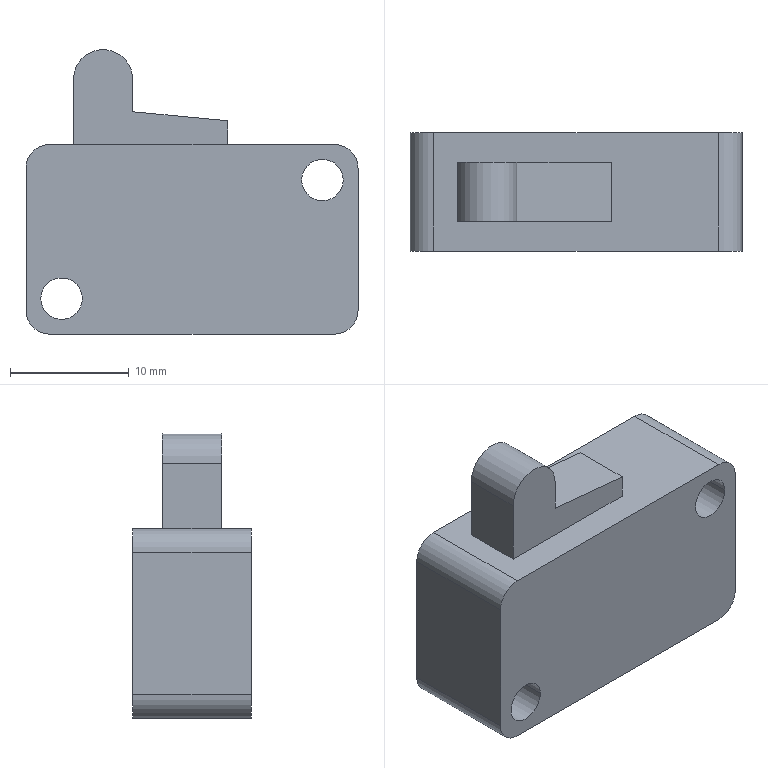Component | SolidWorks | 6G-LimitSwitch-1 | 1 solid | 21 faces | box 28 x 10 x 24 mm | volume 4535 mm3 | plane 12 | cylinder 9 | commonest cylinder face diameters 3.5 x4 4 x4 5 x1
build123d program:
from build123d import *

# Parameters (mm, degrees)
BOSS_EXTRUDE1_DEPTH = 5
SKETCH2_R           = 1.75
CUT_EXTRUDE1_DEPTH  = 10
SKETCH3_W           = 13
SKETCH3_H           = 5
BOSS_EXTRUDE2_DEPTH = 8
CUT_EXTRUDE2_DEPTH  = 8


with BuildPart() as part:
    # Sketch1 → Boss-Extrude1 (new, symmetric)
    with BuildSketch(Plane.XY):
        with BuildLine():
            Line((-12, -8), (12, -8))
            ThreePointArc((12, -8), (13.414, -7.414), (14, -6))
            Line((14, -6), (14, 6))
            ThreePointArc((14, 6), (13.414, 7.414), (12, 8))
            Line((12, 8), (-12, 8))
            ThreePointArc((-12, 8), (-13.414, 7.414), (-14, 6))
            Line((-14, 6), (-14, -6))
            ThreePointArc((-14, -6), (-13.414, -7.414), (-12, -8))
        make_face()
    extrude(amount=BOSS_EXTRUDE1_DEPTH, both=True)

    # Sketch2 → Cut-Extrude1 (cut)
    with BuildSketch(Plane.XY.offset(5)):
        with Locations((-11, 5)):
            Circle(SKETCH2_R)
        with Locations((11, -5)):
            Circle(SKETCH2_R)
    extrude(amount=-CUT_EXTRUDE1_DEPTH, mode=Mode.SUBTRACT)

    # Sketch3 → Boss-Extrude2 (add)
    with BuildSketch(Plane(origin=(0, 8, 0), x_dir=(1, 0, 0), z_dir=(0, 1, 0))):
        with Locations((3.5, 0)):
            Rectangle(SKETCH3_W, SKETCH3_H)
    extrude(amount=BOSS_EXTRUDE2_DEPTH)

    # Sketch4 → Cut-Extrude2 (cut)
    with BuildSketch(Plane.XY.offset(2.5)):
        with BuildLine():
            Line((-3, 10), (5, 10.762))
            Line((5, 10.762), (5, 13.5))
            ThreePointArc((5, 13.5), (7.5, 16), (10, 13.5))
            Line((10, 13.5), (11.275, 13.5))
            Line((11.275, 13.5), (11.275, 18.032))
            Line((11.275, 18.032), (-7.09, 18.279))
            Line((-7.09, 18.279), (-5.465, 11.216))
            Line((-5.465, 11.216), (-3, 10))
        make_face()
    extrude(amount=-CUT_EXTRUDE2_DEPTH, mode=Mode.SUBTRACT)


solid = part.part

# Placed as in the assembly
solid = solid.moved(Location((-161.85, 76, 22), (-90, 0, 180)))
STEP:
#1=COLOUR_RGB('',0.7922,0.8196,0.9333);
#2=FILL_AREA_STYLE_COLOUR('',#1);
#3=FILL_AREA_STYLE('',(#2));
#4=SURFACE_STYLE_FILL_AREA(#3);
#5=SURFACE_SIDE_STYLE('',(#4));
#6=SURFACE_STYLE_USAGE(.BOTH.,#5);
#7=PRESENTATION_STYLE_ASSIGNMENT((#6));
#8=CARTESIAN_POINT('',(-6.736,2.795,0.6693));
#9=VERTEX_POINT('',#8);
#10=CARTESIAN_POINT('',(-6.874,2.795,0.6693));
#11=VERTEX_POINT('',#10);
#12=CARTESIAN_POINT('',(-6.805,2.795,0.6693));
#13=DIRECTION('',(-0.,1.,0.));
#14=DIRECTION('',(-1.,0.,0.));
#15=AXIS2_PLACEMENT_3D('',#12,#13,#14);
#16=CIRCLE('',#15,0.0689);
#17=EDGE_CURVE('',#9,#11,#16,.T.);
#18=ORIENTED_EDGE('',*,*,#17,.F.);
#19=CARTESIAN_POINT('',(-6.736,3.189,0.6693));
#20=VERTEX_POINT('',#19);
#21=CARTESIAN_POINT('',(-6.736,2.795,0.6693));
#22=DIRECTION('',(-0.,1.,0.));
#23=VECTOR('',#22,39.37);
#24=LINE('',#21,#23);
#25=EDGE_CURVE('',#9,#20,#24,.T.);
#26=ORIENTED_EDGE('',*,*,#25,.T.);
#27=CARTESIAN_POINT('',(-6.874,3.189,0.6693));
#28=VERTEX_POINT('',#27);
#29=CARTESIAN_POINT('',(-6.805,3.189,0.6693));
#30=DIRECTION('',(-0.,1.,0.));
#31=DIRECTION('',(-1.,0.,0.));
#32=AXIS2_PLACEMENT_3D('',#29,#30,#31);
#33=CIRCLE('',#32,0.0689);
#34=EDGE_CURVE('',#20,#28,#33,.T.);
#35=ORIENTED_EDGE('',*,*,#34,.T.);
#36=CARTESIAN_POINT('',(-6.874,2.795,0.6693));
#37=DIRECTION('',(-0.,1.,0.));
#38=VECTOR('',#37,39.37);
#39=LINE('',#36,#38);
#40=EDGE_CURVE('',#11,#28,#39,.T.);
#41=ORIENTED_EDGE('',*,*,#40,.F.);
#42=EDGE_LOOP('',(#18,#26,#35,#41));
#43=FACE_OUTER_BOUND('',#42,.T.);
#44=CARTESIAN_POINT('',(-6.805,2.795,0.6693));
#45=DIRECTION('',(-0.,1.,0.));
#46=DIRECTION('',(-1.,0.,0.));
#47=AXIS2_PLACEMENT_3D('',#44,#45,#46);
#48=CYLINDRICAL_SURFACE('',#47,0.0689);
#49=ADVANCED_FACE('',(#43),#48,.F.);
#50=CARTESIAN_POINT('',(-5.87,2.795,1.063));
#51=VERTEX_POINT('',#50);
#52=CARTESIAN_POINT('',(-6.008,2.795,1.063));
#53=VERTEX_POINT('',#52);
#54=CARTESIAN_POINT('',(-5.939,2.795,1.063));
#55=DIRECTION('',(-0.,1.,0.));
#56=DIRECTION('',(-1.,0.,0.));
#57=AXIS2_PLACEMENT_3D('',#54,#55,#56);
#58=CIRCLE('',#57,0.0689);
#59=EDGE_CURVE('',#51,#53,#58,.T.);
#60=ORIENTED_EDGE('',*,*,#59,.F.);
#61=CARTESIAN_POINT('',(-5.87,3.189,1.063));
#62=VERTEX_POINT('',#61);
#63=CARTESIAN_POINT('',(-5.87,2.795,1.063));
#64=DIRECTION('',(-0.,1.,0.));
#65=VECTOR('',#64,39.37);
#66=LINE('',#63,#65);
#67=EDGE_CURVE('',#51,#62,#66,.T.);
#68=ORIENTED_EDGE('',*,*,#67,.T.);
#69=CARTESIAN_POINT('',(-6.008,3.189,1.063));
#70=VERTEX_POINT('',#69);
#71=CARTESIAN_POINT('',(-5.939,3.189,1.063));
#72=DIRECTION('',(-0.,1.,0.));
#73=DIRECTION('',(-1.,0.,0.));
#74=AXIS2_PLACEMENT_3D('',#71,#72,#73);
#75=CIRCLE('',#74,0.0689);
#76=EDGE_CURVE('',#62,#70,#75,.T.);
#77=ORIENTED_EDGE('',*,*,#76,.T.);
#78=CARTESIAN_POINT('',(-6.008,2.795,1.063));
#79=DIRECTION('',(-0.,1.,0.));
#80=VECTOR('',#79,39.37);
#81=LINE('',#78,#80);
#82=EDGE_CURVE('',#53,#70,#81,.T.);
#83=ORIENTED_EDGE('',*,*,#82,.F.);
#84=EDGE_LOOP('',(#60,#68,#77,#83));
#85=FACE_OUTER_BOUND('',#84,.T.);
#86=CARTESIAN_POINT('',(-5.939,2.795,1.063));
#87=DIRECTION('',(-0.,1.,0.));
#88=DIRECTION('',(-1.,0.,0.));
#89=AXIS2_PLACEMENT_3D('',#86,#87,#88);
#90=CYLINDRICAL_SURFACE('',#89,0.0689);
#91=ADVANCED_FACE('',(#85),#90,.F.);
#92=CARTESIAN_POINT('',(-6.844,2.795,1.181));
#93=VERTEX_POINT('',#92);
#94=CARTESIAN_POINT('',(-5.9,2.795,1.181));
#95=VERTEX_POINT('',#94);
#96=CARTESIAN_POINT('',(-5.9,2.795,1.181));
#97=DIRECTION('',(1.,0.,0.));
#98=VECTOR('',#97,39.37);
#99=LINE('',#96,#98);
#100=EDGE_CURVE('',#93,#95,#99,.T.);
#101=ORIENTED_EDGE('',*,*,#100,.T.);
#102=CARTESIAN_POINT('',(-5.9,3.189,1.181));
#103=VERTEX_POINT('',#102);
#104=CARTESIAN_POINT('',(-5.9,3.189,1.181));
#105=DIRECTION('',(0.,-1.,-0.));
#106=VECTOR('',#105,39.37);
#107=LINE('',#104,#106);
#108=EDGE_CURVE('',#103,#95,#107,.T.);
#109=ORIENTED_EDGE('',*,*,#108,.F.);
#110=CARTESIAN_POINT('',(-6.844,3.189,1.181));
#111=VERTEX_POINT('',#110);
#112=CARTESIAN_POINT('',(-5.9,3.189,1.181));
#113=DIRECTION('',(1.,0.,0.));
#114=VECTOR('',#113,39.37);
#115=LINE('',#112,#114);
#116=EDGE_CURVE('',#111,#103,#115,.T.);
#117=ORIENTED_EDGE('',*,*,#116,.F.);
#118=CARTESIAN_POINT('',(-6.844,3.189,1.181));
#119=DIRECTION('',(0.,-1.,-0.));
#120=VECTOR('',#119,39.37);
#121=LINE('',#118,#120);
#122=EDGE_CURVE('',#111,#93,#121,.T.);
#123=ORIENTED_EDGE('',*,*,#122,.T.);
#124=EDGE_LOOP('',(#101,#109,#117,#123));
#125=FACE_OUTER_BOUND('',#124,.T.);
#126=CARTESIAN_POINT('',(-6.766,2.894,1.181));
#127=VERTEX_POINT('',#126);
#128=CARTESIAN_POINT('',(-6.254,2.894,1.181));
#129=VERTEX_POINT('',#128);
#130=CARTESIAN_POINT('',(-6.766,2.894,1.181));
#131=DIRECTION('',(1.,0.,0.));
#132=VECTOR('',#131,39.37);
#133=LINE('',#130,#132);
#134=EDGE_CURVE('',#127,#129,#133,.T.);
#135=ORIENTED_EDGE('',*,*,#134,.F.);
#136=CARTESIAN_POINT('',(-6.766,3.091,1.181));
#137=VERTEX_POINT('',#136);
#138=CARTESIAN_POINT('',(-6.766,3.091,1.181));
#139=DIRECTION('',(0.,-1.,-0.));
#140=VECTOR('',#139,39.37);
#141=LINE('',#138,#140);
#142=EDGE_CURVE('',#137,#127,#141,.T.);
#143=ORIENTED_EDGE('',*,*,#142,.F.);
#144=CARTESIAN_POINT('',(-6.254,3.091,1.181));
#145=VERTEX_POINT('',#144);
#146=CARTESIAN_POINT('',(-6.766,3.091,1.181));
#147=DIRECTION('',(-1.,-0.,-0.));
#148=VECTOR('',#147,39.37);
#149=LINE('',#146,#148);
#150=EDGE_CURVE('',#145,#137,#149,.T.);
#151=ORIENTED_EDGE('',*,*,#150,.F.);
#152=CARTESIAN_POINT('',(-6.254,3.091,1.181));
#153=DIRECTION('',(-0.,1.,0.));
#154=VECTOR('',#153,39.37);
#155=LINE('',#152,#154);
#156=EDGE_CURVE('',#129,#145,#155,.T.);
#157=ORIENTED_EDGE('',*,*,#156,.F.);
#158=EDGE_LOOP('',(#135,#143,#151,#157));
#159=FACE_BOUND('',#158,.T.);
#160=CARTESIAN_POINT('',(-5.9,3.189,1.181));
#161=DIRECTION('',(0.,0.,-1.));
#162=DIRECTION('',(0.,-1.,-0.));
#163=AXIS2_PLACEMENT_3D('',#160,#161,#162);
#164=PLANE('',#163);
#165=ADVANCED_FACE('',(#125,#159),#164,.F.);
#166=CARTESIAN_POINT('',(-5.821,2.795,0.6299));
#167=VERTEX_POINT('',#166);
#168=CARTESIAN_POINT('',(-5.9,2.795,0.5512));
#169=VERTEX_POINT('',#168);
#170=CARTESIAN_POINT('',(-5.9,2.795,0.6299));
#171=DIRECTION('',(-0.,1.,0.));
#172=DIRECTION('',(1.,0.,0.));
#173=AXIS2_PLACEMENT_3D('',#170,#171,#172);
#174=CIRCLE('',#173,0.07874);
#175=EDGE_CURVE('',#167,#169,#174,.T.);
#176=ORIENTED_EDGE('',*,*,#175,.T.);
#177=CARTESIAN_POINT('',(-5.9,3.189,0.5512));
#178=VERTEX_POINT('',#177);
#179=CARTESIAN_POINT('',(-5.9,3.189,0.5512));
#180=DIRECTION('',(0.,-1.,-0.));
#181=VECTOR('',#180,39.37);
#182=LINE('',#179,#181);
#183=EDGE_CURVE('',#178,#169,#182,.T.);
#184=ORIENTED_EDGE('',*,*,#183,.F.);
#185=CARTESIAN_POINT('',(-5.821,3.189,0.6299));
#186=VERTEX_POINT('',#185);
#187=CARTESIAN_POINT('',(-5.9,3.189,0.6299));
#188=DIRECTION('',(-0.,1.,0.));
#189=DIRECTION('',(1.,0.,0.));
#190=AXIS2_PLACEMENT_3D('',#187,#188,#189);
#191=CIRCLE('',#190,0.07874);
#192=EDGE_CURVE('',#186,#178,#191,.T.);
#193=ORIENTED_EDGE('',*,*,#192,.F.);
#194=CARTESIAN_POINT('',(-5.821,3.189,0.6299));
#195=DIRECTION('',(0.,-1.,-0.));
#196=VECTOR('',#195,39.37);
#197=LINE('',#194,#196);
#198=EDGE_CURVE('',#186,#167,#197,.T.);
#199=ORIENTED_EDGE('',*,*,#198,.T.);
#200=EDGE_LOOP('',(#176,#184,#193,#199));
#201=FACE_OUTER_BOUND('',#200,.T.);
#202=CARTESIAN_POINT('',(-5.9,3.189,0.6299));
#203=DIRECTION('',(0.,-1.,-0.));
#204=DIRECTION('',(1.,0.,0.));
#205=AXIS2_PLACEMENT_3D('',#202,#203,#204);
#206=CYLINDRICAL_SURFACE('',#205,0.07874);
#207=ADVANCED_FACE('',(#201),#206,.T.);
#208=CARTESIAN_POINT('',(-6.844,2.795,0.5512));
#209=VERTEX_POINT('',#208);
#210=CARTESIAN_POINT('',(-5.9,2.795,0.5512));
#211=DIRECTION('',(-1.,-0.,-0.));
#212=VECTOR('',#211,39.37);
#213=LINE('',#210,#212);
#214=EDGE_CURVE('',#169,#209,#213,.T.);
#215=ORIENTED_EDGE('',*,*,#214,.T.);
#216=CARTESIAN_POINT('',(-6.844,3.189,0.5512));
#217=VERTEX_POINT('',#216);
#218=CARTESIAN_POINT('',(-6.844,3.189,0.5512));
#219=DIRECTION('',(0.,-1.,-0.));
#220=VECTOR('',#219,39.37);
#221=LINE('',#218,#220);
#222=EDGE_CURVE('',#217,#209,#221,.T.);
#223=ORIENTED_EDGE('',*,*,#222,.F.);
#224=CARTESIAN_POINT('',(-5.9,3.189,0.5512));
#225=DIRECTION('',(-1.,-0.,-0.));
#226=VECTOR('',#225,39.37);
#227=LINE('',#224,#226);
#228=EDGE_CURVE('',#178,#217,#227,.T.);
#229=ORIENTED_EDGE('',*,*,#228,.F.);
#230=ORIENTED_EDGE('',*,*,#183,.T.);
#231=EDGE_LOOP('',(#215,#223,#229,#230));
#232=FACE_OUTER_BOUND('',#231,.T.);
#233=CARTESIAN_POINT('',(-5.9,3.189,0.5512));
#234=DIRECTION('',(-0.,-0.,1.));
#235=DIRECTION('',(-0.,1.,0.));
#236=AXIS2_PLACEMENT_3D('',#233,#234,#235);
#237=PLANE('',#236);
#238=ADVANCED_FACE('',(#232),#237,.F.);
#239=CARTESIAN_POINT('',(-6.923,2.795,0.6299));
#240=VERTEX_POINT('',#239);
#241=CARTESIAN_POINT('',(-6.844,2.795,0.6299));
#242=DIRECTION('',(-0.,1.,0.));
#243=DIRECTION('',(-1.,0.,0.));
#244=AXIS2_PLACEMENT_3D('',#241,#242,#243);
#245=CIRCLE('',#244,0.07874);
#246=EDGE_CURVE('',#209,#240,#245,.T.);
#247=ORIENTED_EDGE('',*,*,#246,.T.);
#248=CARTESIAN_POINT('',(-6.923,3.189,0.6299));
#249=VERTEX_POINT('',#248);
#250=CARTESIAN_POINT('',(-6.923,3.189,0.6299));
#251=DIRECTION('',(0.,-1.,-0.));
#252=VECTOR('',#251,39.37);
#253=LINE('',#250,#252);
#254=EDGE_CURVE('',#249,#240,#253,.T.);
#255=ORIENTED_EDGE('',*,*,#254,.F.);
#256=CARTESIAN_POINT('',(-6.844,3.189,0.6299));
#257=DIRECTION('',(-0.,1.,0.));
#258=DIRECTION('',(-1.,0.,0.));
#259=AXIS2_PLACEMENT_3D('',#256,#257,#258);
#260=CIRCLE('',#259,0.07874);
#261=EDGE_CURVE('',#217,#249,#260,.T.);
#262=ORIENTED_EDGE('',*,*,#261,.F.);
#263=ORIENTED_EDGE('',*,*,#222,.T.);
#264=EDGE_LOOP('',(#247,#255,#262,#263));
#265=FACE_OUTER_BOUND('',#264,.T.);
#266=CARTESIAN_POINT('',(-6.844,3.189,0.6299));
#267=DIRECTION('',(0.,-1.,-0.));
#268=DIRECTION('',(1.,0.,0.));
#269=AXIS2_PLACEMENT_3D('',#266,#267,#268);
#270=CYLINDRICAL_SURFACE('',#269,0.07874);
#271=ADVANCED_FACE('',(#265),#270,.T.);
#272=CARTESIAN_POINT('',(-6.923,2.795,1.102));
#273=VERTEX_POINT('',#272);
#274=CARTESIAN_POINT('',(-6.923,2.795,0.6299));
#275=DIRECTION('',(-0.,-0.,1.));
#276=VECTOR('',#275,39.37);
#277=LINE('',#274,#276);
#278=EDGE_CURVE('',#240,#273,#277,.T.);
#279=ORIENTED_EDGE('',*,*,#278,.T.);
#280=CARTESIAN_POINT('',(-6.923,3.189,1.102));
#281=VERTEX_POINT('',#280);
#282=CARTESIAN_POINT('',(-6.923,3.189,1.102));
#283=DIRECTION('',(0.,-1.,-0.));
#284=VECTOR('',#283,39.37);
#285=LINE('',#282,#284);
#286=EDGE_CURVE('',#281,#273,#285,.T.);
#287=ORIENTED_EDGE('',*,*,#286,.F.);
#288=CARTESIAN_POINT('',(-6.923,3.189,0.6299));
#289=DIRECTION('',(-0.,-0.,1.));
#290=VECTOR('',#289,39.37);
#291=LINE('',#288,#290);
#292=EDGE_CURVE('',#249,#281,#291,.T.);
#293=ORIENTED_EDGE('',*,*,#292,.F.);
#294=ORIENTED_EDGE('',*,*,#254,.T.);
#295=EDGE_LOOP('',(#279,#287,#293,#294));
#296=FACE_OUTER_BOUND('',#295,.T.);
#297=CARTESIAN_POINT('',(-6.923,3.189,0.6299));
#298=DIRECTION('',(1.,0.,0.));
#299=DIRECTION('',(-0.,1.,0.));
#300=AXIS2_PLACEMENT_3D('',#297,#298,#299);
#301=PLANE('',#300);
#302=ADVANCED_FACE('',(#296),#301,.F.);
#303=CARTESIAN_POINT('',(-6.844,2.795,1.102));
#304=DIRECTION('',(-0.,1.,0.));
#305=DIRECTION('',(1.,0.,0.));
#306=AXIS2_PLACEMENT_3D('',#303,#304,#305);
#307=CIRCLE('',#306,0.07874);
#308=EDGE_CURVE('',#273,#93,#307,.T.);
#309=ORIENTED_EDGE('',*,*,#308,.T.);
#310=ORIENTED_EDGE('',*,*,#122,.F.);
#311=CARTESIAN_POINT('',(-6.844,3.189,1.102));
#312=DIRECTION('',(-0.,1.,0.));
#313=DIRECTION('',(1.,0.,0.));
#314=AXIS2_PLACEMENT_3D('',#311,#312,#313);
#315=CIRCLE('',#314,0.07874);
#316=EDGE_CURVE('',#281,#111,#315,.T.);
#317=ORIENTED_EDGE('',*,*,#316,.F.);
#318=ORIENTED_EDGE('',*,*,#286,.T.);
#319=EDGE_LOOP('',(#309,#310,#317,#318));
#320=FACE_OUTER_BOUND('',#319,.T.);
#321=CARTESIAN_POINT('',(-6.844,3.189,1.102));
#322=DIRECTION('',(0.,-1.,-0.));
#323=DIRECTION('',(1.,0.,0.));
#324=AXIS2_PLACEMENT_3D('',#321,#322,#323);
#325=CYLINDRICAL_SURFACE('',#324,0.07874);
#326=ADVANCED_FACE('',(#320),#325,.T.);
#327=CARTESIAN_POINT('',(-5.821,2.795,1.102));
#328=VERTEX_POINT('',#327);
#329=CARTESIAN_POINT('',(-5.9,2.795,1.102));
#330=DIRECTION('',(-0.,1.,0.));
#331=DIRECTION('',(1.,0.,0.));
#332=AXIS2_PLACEMENT_3D('',#329,#330,#331);
#333=CIRCLE('',#332,0.07874);
#334=EDGE_CURVE('',#95,#328,#333,.T.);
#335=ORIENTED_EDGE('',*,*,#334,.T.);
#336=CARTESIAN_POINT('',(-5.821,3.189,1.102));
#337=VERTEX_POINT('',#336);
#338=CARTESIAN_POINT('',(-5.821,3.189,1.102));
#339=DIRECTION('',(0.,-1.,-0.));
#340=VECTOR('',#339,39.37);
#341=LINE('',#338,#340);
#342=EDGE_CURVE('',#337,#328,#341,.T.);
#343=ORIENTED_EDGE('',*,*,#342,.F.);
#344=CARTESIAN_POINT('',(-5.9,3.189,1.102));
#345=DIRECTION('',(-0.,1.,0.));
#346=DIRECTION('',(1.,0.,0.));
#347=AXIS2_PLACEMENT_3D('',#344,#345,#346);
#348=CIRCLE('',#347,0.07874);
#349=EDGE_CURVE('',#103,#337,#348,.T.);
#350=ORIENTED_EDGE('',*,*,#349,.F.);
#351=ORIENTED_EDGE('',*,*,#108,.T.);
#352=EDGE_LOOP('',(#335,#343,#350,#351));
#353=FACE_OUTER_BOUND('',#352,.T.);
#354=CARTESIAN_POINT('',(-5.9,3.189,1.102));
#355=DIRECTION('',(0.,-1.,-0.));
#356=DIRECTION('',(1.,0.,0.));
#357=AXIS2_PLACEMENT_3D('',#354,#355,#356);
#358=CYLINDRICAL_SURFACE('',#357,0.07874);
#359=ADVANCED_FACE('',(#353),#358,.T.);
#360=CARTESIAN_POINT('',(-5.821,2.795,0.6299));
#361=DIRECTION('',(0.,0.,-1.));
#362=VECTOR('',#361,39.37);
#363=LINE('',#360,#362);
#364=EDGE_CURVE('',#328,#167,#363,.T.);
#365=ORIENTED_EDGE('',*,*,#364,.T.);
#366=ORIENTED_EDGE('',*,*,#198,.F.);
#367=CARTESIAN_POINT('',(-5.821,3.189,0.6299));
#368=DIRECTION('',(0.,0.,-1.));
#369=VECTOR('',#368,39.37);
#370=LINE('',#367,#369);
#371=EDGE_CURVE('',#337,#186,#370,.T.);
#372=ORIENTED_EDGE('',*,*,#371,.F.);
#373=ORIENTED_EDGE('',*,*,#342,.T.);
#374=EDGE_LOOP('',(#365,#366,#372,#373));
#375=FACE_OUTER_BOUND('',#374,.T.);
#376=CARTESIAN_POINT('',(-5.821,3.189,0.6299));
#377=DIRECTION('',(-1.,-0.,-0.));
#378=DIRECTION('',(0.,-1.,-0.));
#379=AXIS2_PLACEMENT_3D('',#376,#377,#378);
#380=PLANE('',#379);
#381=ADVANCED_FACE('',(#375),#380,.F.);
#382=CARTESIAN_POINT('',(-6.805,3.189,0.6693));
#383=DIRECTION('',(-0.,1.,0.));
#384=DIRECTION('',(-1.,0.,0.));
#385=AXIS2_PLACEMENT_3D('',#382,#383,#384);
#386=CIRCLE('',#385,0.0689);
#387=EDGE_CURVE('',#28,#20,#386,.T.);
#388=ORIENTED_EDGE('',*,*,#387,.F.);
#389=ORIENTED_EDGE('',*,*,#34,.F.);
#390=EDGE_LOOP('',(#388,#389));
#391=FACE_BOUND('',#390,.T.);
#392=CARTESIAN_POINT('',(-5.939,3.189,1.063));
#393=DIRECTION('',(-0.,1.,0.));
#394=DIRECTION('',(-1.,0.,0.));
#395=AXIS2_PLACEMENT_3D('',#392,#393,#394);
#396=CIRCLE('',#395,0.0689);
#397=EDGE_CURVE('',#70,#62,#396,.T.);
#398=ORIENTED_EDGE('',*,*,#397,.F.);
#399=ORIENTED_EDGE('',*,*,#76,.F.);
#400=EDGE_LOOP('',(#398,#399));
#401=FACE_BOUND('',#400,.T.);
#402=ORIENTED_EDGE('',*,*,#192,.T.);
#403=ORIENTED_EDGE('',*,*,#228,.T.);
#404=ORIENTED_EDGE('',*,*,#261,.T.);
#405=ORIENTED_EDGE('',*,*,#292,.T.);
#406=ORIENTED_EDGE('',*,*,#316,.T.);
#407=ORIENTED_EDGE('',*,*,#116,.T.);
#408=ORIENTED_EDGE('',*,*,#349,.T.);
#409=ORIENTED_EDGE('',*,*,#371,.T.);
#410=EDGE_LOOP('',(#402,#403,#404,#405,#406,#407,#408,#409));
#411=FACE_OUTER_BOUND('',#410,.T.);
#412=CARTESIAN_POINT('',(-5.9,3.189,0.6299));
#413=DIRECTION('',(0.,-1.,-0.));
#414=DIRECTION('',(1.,0.,0.));
#415=AXIS2_PLACEMENT_3D('',#412,#413,#414);
#416=PLANE('',#415);
#417=ADVANCED_FACE('',(#391,#401,#411),#416,.F.);
#418=CARTESIAN_POINT('',(-6.805,2.795,0.6693));
#419=DIRECTION('',(-0.,1.,0.));
#420=DIRECTION('',(-1.,0.,0.));
#421=AXIS2_PLACEMENT_3D('',#418,#419,#420);
#422=CIRCLE('',#421,0.0689);
#423=EDGE_CURVE('',#11,#9,#422,.T.);
#424=ORIENTED_EDGE('',*,*,#423,.T.);
#425=ORIENTED_EDGE('',*,*,#17,.T.);
#426=EDGE_LOOP('',(#424,#425));
#427=FACE_BOUND('',#426,.T.);
#428=CARTESIAN_POINT('',(-5.939,2.795,1.063));
#429=DIRECTION('',(-0.,1.,0.));
#430=DIRECTION('',(-1.,0.,0.));
#431=AXIS2_PLACEMENT_3D('',#428,#429,#430);
#432=CIRCLE('',#431,0.0689);
#433=EDGE_CURVE('',#53,#51,#432,.T.);
#434=ORIENTED_EDGE('',*,*,#433,.T.);
#435=ORIENTED_EDGE('',*,*,#59,.T.);
#436=EDGE_LOOP('',(#434,#435));
#437=FACE_BOUND('',#436,.T.);
#438=ORIENTED_EDGE('',*,*,#175,.F.);
#439=ORIENTED_EDGE('',*,*,#364,.F.);
#440=ORIENTED_EDGE('',*,*,#334,.F.);
#441=ORIENTED_EDGE('',*,*,#100,.F.);
#442=ORIENTED_EDGE('',*,*,#308,.F.);
#443=ORIENTED_EDGE('',*,*,#278,.F.);
#444=ORIENTED_EDGE('',*,*,#246,.F.);
#445=ORIENTED_EDGE('',*,*,#214,.F.);
#446=EDGE_LOOP('',(#438,#439,#440,#441,#442,#443,#444,#445));
#447=FACE_OUTER_BOUND('',#446,.T.);
#448=CARTESIAN_POINT('',(-5.9,2.795,0.6299));
#449=DIRECTION('',(0.,-1.,-0.));
#450=DIRECTION('',(1.,0.,0.));
#451=AXIS2_PLACEMENT_3D('',#448,#449,#450);
#452=PLANE('',#451);
#453=ADVANCED_FACE('',(#427,#437,#447),#452,.T.);
#454=ORIENTED_EDGE('',*,*,#67,.F.);
#455=ORIENTED_EDGE('',*,*,#433,.F.);
#456=ORIENTED_EDGE('',*,*,#82,.T.);
#457=ORIENTED_EDGE('',*,*,#397,.T.);
#458=EDGE_LOOP('',(#454,#455,#456,#457));
#459=FACE_OUTER_BOUND('',#458,.T.);
#460=CARTESIAN_POINT('',(-5.939,2.795,1.063));
#461=DIRECTION('',(-0.,1.,0.));
#462=DIRECTION('',(-1.,0.,0.));
#463=AXIS2_PLACEMENT_3D('',#460,#461,#462);
#464=CYLINDRICAL_SURFACE('',#463,0.0689);
#465=ADVANCED_FACE('',(#459),#464,.F.);
#466=ORIENTED_EDGE('',*,*,#25,.F.);
#467=ORIENTED_EDGE('',*,*,#423,.F.);
#468=ORIENTED_EDGE('',*,*,#40,.T.);
#469=ORIENTED_EDGE('',*,*,#387,.T.);
#470=EDGE_LOOP('',(#466,#467,#468,#469));
#471=FACE_OUTER_BOUND('',#470,.T.);
#472=CARTESIAN_POINT('',(-6.805,2.795,0.6693));
#473=DIRECTION('',(-0.,1.,0.));
#474=DIRECTION('',(-1.,0.,0.));
#475=AXIS2_PLACEMENT_3D('',#472,#473,#474);
#476=CYLINDRICAL_SURFACE('',#475,0.0689);
#477=ADVANCED_FACE('',(#471),#476,.F.);
#478=CARTESIAN_POINT('',(-6.569,2.894,1.398));
#479=VERTEX_POINT('',#478);
#480=CARTESIAN_POINT('',(-6.766,2.894,1.398));
#481=VERTEX_POINT('',#480);
#482=CARTESIAN_POINT('',(-6.667,2.894,1.398));
#483=DIRECTION('',(0.,-1.,-0.));
#484=DIRECTION('',(-1.,0.,0.));
#485=AXIS2_PLACEMENT_3D('',#482,#483,#484);
#486=CIRCLE('',#485,0.09843);
#487=EDGE_CURVE('',#479,#481,#486,.T.);
#488=ORIENTED_EDGE('',*,*,#487,.T.);
#489=CARTESIAN_POINT('',(-6.766,2.894,1.496));
#490=DIRECTION('',(0.,0.,-1.));
#491=VECTOR('',#490,39.37);
#492=LINE('',#489,#491);
#493=EDGE_CURVE('',#481,#127,#492,.T.);
#494=ORIENTED_EDGE('',*,*,#493,.T.);
#495=ORIENTED_EDGE('',*,*,#134,.T.);
#496=CARTESIAN_POINT('',(-6.254,2.894,1.26));
#497=VERTEX_POINT('',#496);
#498=CARTESIAN_POINT('',(-6.254,2.894,1.496));
#499=DIRECTION('',(0.,0.,-1.));
#500=VECTOR('',#499,39.37);
#501=LINE('',#498,#500);
#502=EDGE_CURVE('',#497,#129,#501,.T.);
#503=ORIENTED_EDGE('',*,*,#502,.F.);
#504=CARTESIAN_POINT('',(-6.569,2.894,1.29));
#505=VERTEX_POINT('',#504);
#506=CARTESIAN_POINT('',(-6.783,2.894,1.31));
#507=DIRECTION('',(-0.9955,-0.,0.09481));
#508=VECTOR('',#507,39.37);
#509=LINE('',#506,#508);
#510=EDGE_CURVE('',#497,#505,#509,.T.);
#511=ORIENTED_EDGE('',*,*,#510,.T.);
#512=CARTESIAN_POINT('',(-6.569,2.894,1.496));
#513=DIRECTION('',(-0.,-0.,1.));
#514=VECTOR('',#513,39.37);
#515=LINE('',#512,#514);
#516=EDGE_CURVE('',#505,#479,#515,.T.);
#517=ORIENTED_EDGE('',*,*,#516,.T.);
#518=EDGE_LOOP('',(#488,#494,#495,#503,#511,#517));
#519=FACE_OUTER_BOUND('',#518,.T.);
#520=CARTESIAN_POINT('',(-6.766,2.894,1.496));
#521=DIRECTION('',(-0.,1.,0.));
#522=DIRECTION('',(-1.,-0.,-0.));
#523=AXIS2_PLACEMENT_3D('',#520,#521,#522);
#524=PLANE('',#523);
#525=ADVANCED_FACE('',(#519),#524,.F.);
#526=CARTESIAN_POINT('',(-6.254,3.091,1.26));
#527=VERTEX_POINT('',#526);
#528=CARTESIAN_POINT('',(-6.254,3.091,1.496));
#529=DIRECTION('',(0.,0.,-1.));
#530=VECTOR('',#529,39.37);
#531=LINE('',#528,#530);
#532=EDGE_CURVE('',#527,#145,#531,.T.);
#533=ORIENTED_EDGE('',*,*,#532,.F.);
#534=CARTESIAN_POINT('',(-6.254,2.776,1.26));
#535=DIRECTION('',(-0.,1.,0.));
#536=VECTOR('',#535,39.37);
#537=LINE('',#534,#536);
#538=EDGE_CURVE('',#497,#527,#537,.T.);
#539=ORIENTED_EDGE('',*,*,#538,.F.);
#540=ORIENTED_EDGE('',*,*,#502,.T.);
#541=ORIENTED_EDGE('',*,*,#156,.T.);
#542=EDGE_LOOP('',(#533,#539,#540,#541));
#543=FACE_OUTER_BOUND('',#542,.T.);
#544=CARTESIAN_POINT('',(-6.254,3.091,1.496));
#545=DIRECTION('',(-1.,-0.,-0.));
#546=DIRECTION('',(0.,-1.,-0.));
#547=AXIS2_PLACEMENT_3D('',#544,#545,#546);
#548=PLANE('',#547);
#549=ADVANCED_FACE('',(#543),#548,.F.);
#550=CARTESIAN_POINT('',(-6.766,3.091,1.398));
#551=VERTEX_POINT('',#550);
#552=CARTESIAN_POINT('',(-6.766,3.091,1.496));
#553=DIRECTION('',(0.,0.,-1.));
#554=VECTOR('',#553,39.37);
#555=LINE('',#552,#554);
#556=EDGE_CURVE('',#551,#137,#555,.T.);
#557=ORIENTED_EDGE('',*,*,#556,.F.);
#558=CARTESIAN_POINT('',(-6.569,3.091,1.398));
#559=VERTEX_POINT('',#558);
#560=CARTESIAN_POINT('',(-6.667,3.091,1.398));
#561=DIRECTION('',(0.,-1.,-0.));
#562=DIRECTION('',(-1.,0.,0.));
#563=AXIS2_PLACEMENT_3D('',#560,#561,#562);
#564=CIRCLE('',#563,0.09843);
#565=EDGE_CURVE('',#559,#551,#564,.T.);
#566=ORIENTED_EDGE('',*,*,#565,.F.);
#567=CARTESIAN_POINT('',(-6.569,3.091,1.29));
#568=VERTEX_POINT('',#567);
#569=CARTESIAN_POINT('',(-6.569,3.091,1.398));
#570=DIRECTION('',(-0.,-0.,1.));
#571=VECTOR('',#570,39.37);
#572=LINE('',#569,#571);
#573=EDGE_CURVE('',#568,#559,#572,.T.);
#574=ORIENTED_EDGE('',*,*,#573,.F.);
#575=CARTESIAN_POINT('',(-6.254,3.091,1.26));
#576=DIRECTION('',(-0.9955,-0.,0.09481));
#577=VECTOR('',#576,39.37);
#578=LINE('',#575,#577);
#579=EDGE_CURVE('',#527,#568,#578,.T.);
#580=ORIENTED_EDGE('',*,*,#579,.F.);
#581=ORIENTED_EDGE('',*,*,#532,.T.);
#582=ORIENTED_EDGE('',*,*,#150,.T.);
#583=EDGE_LOOP('',(#557,#566,#574,#580,#581,#582));
#584=FACE_OUTER_BOUND('',#583,.T.);
#585=CARTESIAN_POINT('',(-6.766,3.091,1.496));
#586=DIRECTION('',(0.,-1.,-0.));
#587=DIRECTION('',(1.,0.,0.));
#588=AXIS2_PLACEMENT_3D('',#585,#586,#587);
#589=PLANE('',#588);
#590=ADVANCED_FACE('',(#584),#589,.F.);
#591=ORIENTED_EDGE('',*,*,#493,.F.);
#592=CARTESIAN_POINT('',(-6.766,2.776,1.398));
#593=DIRECTION('',(-0.,1.,0.));
#594=VECTOR('',#593,39.37);
#595=LINE('',#592,#594);
#596=EDGE_CURVE('',#481,#551,#595,.T.);
#597=ORIENTED_EDGE('',*,*,#596,.T.);
#598=ORIENTED_EDGE('',*,*,#556,.T.);
#599=ORIENTED_EDGE('',*,*,#142,.T.);
#600=EDGE_LOOP('',(#591,#597,#598,#599));
#601=FACE_OUTER_BOUND('',#600,.T.);
#602=CARTESIAN_POINT('',(-6.766,3.091,1.496));
#603=DIRECTION('',(1.,0.,0.));
#604=DIRECTION('',(-0.,1.,0.));
#605=AXIS2_PLACEMENT_3D('',#602,#603,#604);
#606=PLANE('',#605);
#607=ADVANCED_FACE('',(#601),#606,.F.);
#608=CARTESIAN_POINT('',(-6.569,2.776,1.29));
#609=DIRECTION('',(-0.,1.,0.));
#610=VECTOR('',#609,39.37);
#611=LINE('',#608,#610);
#612=EDGE_CURVE('',#505,#568,#611,.T.);
#613=ORIENTED_EDGE('',*,*,#612,.T.);
#614=ORIENTED_EDGE('',*,*,#573,.T.);
#615=CARTESIAN_POINT('',(-6.569,2.776,1.398));
#616=DIRECTION('',(-0.,1.,0.));
#617=VECTOR('',#616,39.37);
#618=LINE('',#615,#617);
#619=EDGE_CURVE('',#479,#559,#618,.T.);
#620=ORIENTED_EDGE('',*,*,#619,.F.);
#621=ORIENTED_EDGE('',*,*,#516,.F.);
#622=EDGE_LOOP('',(#613,#614,#620,#621));
#623=FACE_OUTER_BOUND('',#622,.T.);
#624=CARTESIAN_POINT('',(-6.569,2.776,1.398));
#625=DIRECTION('',(-1.,-0.,-0.));
#626=DIRECTION('',(0.,-1.,-0.));
#627=AXIS2_PLACEMENT_3D('',#624,#625,#626);
#628=PLANE('',#627);
#629=ADVANCED_FACE('',(#623),#628,.F.);
#630=ORIENTED_EDGE('',*,*,#538,.T.);
#631=ORIENTED_EDGE('',*,*,#579,.T.);
#632=ORIENTED_EDGE('',*,*,#612,.F.);
#633=ORIENTED_EDGE('',*,*,#510,.F.);
#634=EDGE_LOOP('',(#630,#631,#632,#633));
#635=FACE_OUTER_BOUND('',#634,.T.);
#636=CARTESIAN_POINT('',(-6.254,2.776,1.26));
#637=DIRECTION('',(-0.09481,-0.,-0.9955));
#638=DIRECTION('',(-0.9955,-0.,0.09481));
#639=AXIS2_PLACEMENT_3D('',#636,#637,#638);
#640=PLANE('',#639);
#641=ADVANCED_FACE('',(#635),#640,.F.);
#642=ORIENTED_EDGE('',*,*,#619,.T.);
#643=ORIENTED_EDGE('',*,*,#565,.T.);
#644=ORIENTED_EDGE('',*,*,#596,.F.);
#645=ORIENTED_EDGE('',*,*,#487,.F.);
#646=EDGE_LOOP('',(#642,#643,#644,#645));
#647=FACE_OUTER_BOUND('',#646,.T.);
#648=CARTESIAN_POINT('',(-6.667,2.776,1.398));
#649=DIRECTION('',(-0.,1.,0.));
#650=DIRECTION('',(-1.,0.,0.));
#651=AXIS2_PLACEMENT_3D('',#648,#649,#650);
#652=CYLINDRICAL_SURFACE('',#651,0.09843);
#653=ADVANCED_FACE('',(#647),#652,.T.);
#654=CLOSED_SHELL('',(#49,#91,#165,#207,#238,#271,#302,#326,#359,#381,#417,#453,#465,#477,#525,#549,#590,#607,#629,#641,#653));
#655=MANIFOLD_SOLID_BREP('',#654);
#656=STYLED_ITEM('',(#7),#655);
#657=(LENGTH_UNIT()NAMED_UNIT(*)SI_UNIT($,.METRE.));
#658=LENGTH_MEASURE_WITH_UNIT(LENGTH_MEASURE(0.0254),#657);
#659=DIMENSIONAL_EXPONENTS(1.,0.,0.,0.,0.,0.,0.);
#660=(CONVERSION_BASED_UNIT('',#658)LENGTH_UNIT()NAMED_UNIT(#659));
#661=UNCERTAINTY_MEASURE_WITH_UNIT(LENGTH_MEASURE(0.00001),#660,'','');
#662=(NAMED_UNIT(*)PLANE_ANGLE_UNIT()SI_UNIT($,.RADIAN.));
#663=(NAMED_UNIT(*)SI_UNIT($,.STERADIAN.)SOLID_ANGLE_UNIT());
#664=(GEOMETRIC_REPRESENTATION_CONTEXT(3)GLOBAL_UNCERTAINTY_ASSIGNED_CONTEXT((#661))GLOBAL_UNIT_ASSIGNED_CONTEXT((#660,#662,#663))REPRESENTATION_CONTEXT('',''));
#665=MECHANICAL_DESIGN_GEOMETRIC_PRESENTATION_REPRESENTATION('',(#656),#664);
#666=CARTESIAN_POINT('',(0.,0.,0.));
#667=DIRECTION('',(0.,0.,1.));
#668=DIRECTION('',(1.,0.,0.));
#669=AXIS2_PLACEMENT_3D('',#666,#667,#668);
#670=(LENGTH_UNIT()NAMED_UNIT(*)SI_UNIT($,.METRE.));
#671=LENGTH_MEASURE_WITH_UNIT(LENGTH_MEASURE(0.0254),#670);
#672=DIMENSIONAL_EXPONENTS(1.,0.,0.,0.,0.,0.,0.);
#673=(CONVERSION_BASED_UNIT('',#671)LENGTH_UNIT()NAMED_UNIT(#672));
#674=UNCERTAINTY_MEASURE_WITH_UNIT(LENGTH_MEASURE(0.00001),#673,'','');
#675=(NAMED_UNIT(*)PLANE_ANGLE_UNIT()SI_UNIT($,.RADIAN.));
#676=(NAMED_UNIT(*)SI_UNIT($,.STERADIAN.)SOLID_ANGLE_UNIT());
#677=(GEOMETRIC_REPRESENTATION_CONTEXT(3)GLOBAL_UNCERTAINTY_ASSIGNED_CONTEXT((#674))GLOBAL_UNIT_ASSIGNED_CONTEXT((#673,#675,#676))REPRESENTATION_CONTEXT('',''));
#678=ADVANCED_BREP_SHAPE_REPRESENTATION('',(#655,#669),#677);
#679=PRESENTATION_LAYER_ASSIGNMENT('','',(#656));